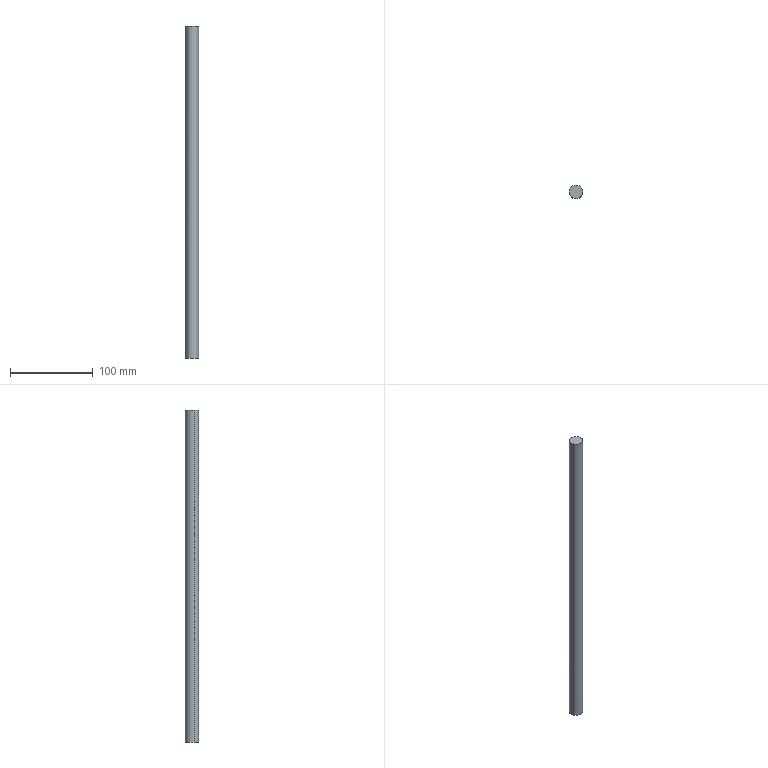Component | SolidWorks | CSFA2082 078-5 | 1 solid | 4 faces | box 16 x 16 x 400 mm | volume 80425 mm3 | cylinder 2 | plane 2 | commonest cylinder face diameters 16 x2
build123d program:
from build123d import *

# Parameters (mm, degrees)
SKETCH1_R      = 8
EXTRUDE1_DEPTH = 400


with BuildPart() as part:
    # Sketch1 → Extrude1 (new body)
    with BuildSketch(Plane.XY):
        Circle(SKETCH1_R)
    extrude(amount=EXTRUDE1_DEPTH)


solid = part.part

# Placed as in the assembly
solid = solid.moved(Location((-337.449, -241.176, 87), (0, 0, 0)))
STEP:
#1=CARTESIAN_POINT('',(-12.989,-9.387,19.173));
#2=VERTEX_POINT('',#1);
#3=CARTESIAN_POINT('',(-13.581,-9.603,19.173));
#4=VERTEX_POINT('',#3);
#5=CARTESIAN_POINT('',(-13.285,-9.495,19.173));
#6=DIRECTION('',(0.,0.,1.));
#7=DIRECTION('',(0.9395,0.3426,0.));
#8=AXIS2_PLACEMENT_3D('',#5,#6,#7);
#9=CIRCLE('',#8,0.315);
#10=EDGE_CURVE('',#2,#4,#9,.T.);
#11=ORIENTED_EDGE('',*,*,#10,.F.);
#12=CARTESIAN_POINT('',(-12.989,-9.387,3.425));
#13=VERTEX_POINT('',#12);
#14=CARTESIAN_POINT('',(-12.989,-9.387,19.173));
#15=DIRECTION('',(0.,0.,-1.));
#16=VECTOR('',#15,39.37);
#17=LINE('',#14,#16);
#18=EDGE_CURVE('',#2,#13,#17,.T.);
#19=ORIENTED_EDGE('',*,*,#18,.T.);
#20=CARTESIAN_POINT('',(-13.581,-9.603,3.425));
#21=VERTEX_POINT('',#20);
#22=CARTESIAN_POINT('',(-13.285,-9.495,3.425));
#23=DIRECTION('',(0.,0.,1.));
#24=DIRECTION('',(0.9395,0.3426,0.));
#25=AXIS2_PLACEMENT_3D('',#22,#23,#24);
#26=CIRCLE('',#25,0.315);
#27=EDGE_CURVE('',#13,#21,#26,.T.);
#28=ORIENTED_EDGE('',*,*,#27,.T.);
#29=CARTESIAN_POINT('',(-13.581,-9.603,19.173));
#30=DIRECTION('',(0.,0.,-1.));
#31=VECTOR('',#30,39.37);
#32=LINE('',#29,#31);
#33=EDGE_CURVE('',#4,#21,#32,.T.);
#34=ORIENTED_EDGE('',*,*,#33,.F.);
#35=EDGE_LOOP('',(#11,#19,#28,#34));
#36=FACE_OUTER_BOUND('',#35,.T.);
#37=CARTESIAN_POINT('',(-13.285,-9.495,19.173));
#38=DIRECTION('',(0.,0.,-1.));
#39=DIRECTION('',(-0.9395,-0.3426,0.));
#40=AXIS2_PLACEMENT_3D('',#37,#38,#39);
#41=CYLINDRICAL_SURFACE('',#40,0.315);
#42=ADVANCED_FACE('',(#36),#41,.T.);
#43=ORIENTED_EDGE('',*,*,#18,.F.);
#44=CARTESIAN_POINT('',(-13.285,-9.495,19.173));
#45=DIRECTION('',(0.,0.,1.));
#46=DIRECTION('',(0.9395,0.3426,0.));
#47=AXIS2_PLACEMENT_3D('',#44,#45,#46);
#48=CIRCLE('',#47,0.315);
#49=EDGE_CURVE('',#4,#2,#48,.T.);
#50=ORIENTED_EDGE('',*,*,#49,.F.);
#51=ORIENTED_EDGE('',*,*,#33,.T.);
#52=CARTESIAN_POINT('',(-13.285,-9.495,3.425));
#53=DIRECTION('',(0.,0.,1.));
#54=DIRECTION('',(0.9395,0.3426,0.));
#55=AXIS2_PLACEMENT_3D('',#52,#53,#54);
#56=CIRCLE('',#55,0.315);
#57=EDGE_CURVE('',#21,#13,#56,.T.);
#58=ORIENTED_EDGE('',*,*,#57,.T.);
#59=EDGE_LOOP('',(#43,#50,#51,#58));
#60=FACE_OUTER_BOUND('',#59,.T.);
#61=CARTESIAN_POINT('',(-13.285,-9.495,19.173));
#62=DIRECTION('',(0.,0.,-1.));
#63=DIRECTION('',(-0.9395,-0.3426,0.));
#64=AXIS2_PLACEMENT_3D('',#61,#62,#63);
#65=CYLINDRICAL_SURFACE('',#64,0.315);
#66=ADVANCED_FACE('',(#60),#65,.T.);
#67=ORIENTED_EDGE('',*,*,#49,.T.);
#68=ORIENTED_EDGE('',*,*,#10,.T.);
#69=EDGE_LOOP('',(#67,#68));
#70=FACE_OUTER_BOUND('',#69,.T.);
#71=CARTESIAN_POINT('',(-13.285,-9.495,19.173));
#72=DIRECTION('',(0.,0.,1.));
#73=DIRECTION('',(0.9395,0.3426,0.));
#74=AXIS2_PLACEMENT_3D('',#71,#72,#73);
#75=PLANE('',#74);
#76=ADVANCED_FACE('',(#70),#75,.T.);
#77=ORIENTED_EDGE('',*,*,#57,.F.);
#78=ORIENTED_EDGE('',*,*,#27,.F.);
#79=EDGE_LOOP('',(#77,#78));
#80=FACE_OUTER_BOUND('',#79,.T.);
#81=CARTESIAN_POINT('',(-13.285,-9.495,3.425));
#82=DIRECTION('',(0.,0.,1.));
#83=DIRECTION('',(0.9395,0.3426,0.));
#84=AXIS2_PLACEMENT_3D('',#81,#82,#83);
#85=PLANE('',#84);
#86=ADVANCED_FACE('',(#80),#85,.F.);
#87=CLOSED_SHELL('',(#42,#66,#76,#86));
#88=MANIFOLD_SOLID_BREP('',#87);
#89=CARTESIAN_POINT('',(0.,0.,0.));
#90=DIRECTION('',(0.,0.,1.));
#91=DIRECTION('',(1.,0.,0.));
#92=AXIS2_PLACEMENT_3D('',#89,#90,#91);
#93=(LENGTH_UNIT()NAMED_UNIT(*)SI_UNIT($,.METRE.));
#94=LENGTH_MEASURE_WITH_UNIT(LENGTH_MEASURE(0.0254),#93);
#95=DIMENSIONAL_EXPONENTS(1.,0.,0.,0.,0.,0.,0.);
#96=(CONVERSION_BASED_UNIT('',#94)LENGTH_UNIT()NAMED_UNIT(#95));
#97=UNCERTAINTY_MEASURE_WITH_UNIT(LENGTH_MEASURE(0.00001),#96,'','');
#98=(NAMED_UNIT(*)PLANE_ANGLE_UNIT()SI_UNIT($,.RADIAN.));
#99=(NAMED_UNIT(*)SI_UNIT($,.STERADIAN.)SOLID_ANGLE_UNIT());
#100=(GEOMETRIC_REPRESENTATION_CONTEXT(3)GLOBAL_UNCERTAINTY_ASSIGNED_CONTEXT((#97))GLOBAL_UNIT_ASSIGNED_CONTEXT((#96,#98,#99))REPRESENTATION_CONTEXT('',''));
#101=ADVANCED_BREP_SHAPE_REPRESENTATION('',(#88,#92),#100);
#102=COLOUR_RGB('',0.7922,0.8196,0.9333);
#103=FILL_AREA_STYLE_COLOUR('',#102);
#104=FILL_AREA_STYLE('',(#103));
#105=SURFACE_STYLE_FILL_AREA(#104);
#106=SURFACE_SIDE_STYLE('',(#105));
#107=SURFACE_STYLE_USAGE(.BOTH.,#106);
#108=PRESENTATION_STYLE_ASSIGNMENT((#107));
#109=STYLED_ITEM('',(#108),#88);
#110=(LENGTH_UNIT()NAMED_UNIT(*)SI_UNIT($,.METRE.));
#111=LENGTH_MEASURE_WITH_UNIT(LENGTH_MEASURE(0.0254),#110);
#112=DIMENSIONAL_EXPONENTS(1.,0.,0.,0.,0.,0.,0.);
#113=(CONVERSION_BASED_UNIT('',#111)LENGTH_UNIT()NAMED_UNIT(#112));
#114=UNCERTAINTY_MEASURE_WITH_UNIT(LENGTH_MEASURE(0.00001),#113,'','');
#115=(NAMED_UNIT(*)PLANE_ANGLE_UNIT()SI_UNIT($,.RADIAN.));
#116=(NAMED_UNIT(*)SI_UNIT($,.STERADIAN.)SOLID_ANGLE_UNIT());
#117=(GEOMETRIC_REPRESENTATION_CONTEXT(3)GLOBAL_UNCERTAINTY_ASSIGNED_CONTEXT((#114))GLOBAL_UNIT_ASSIGNED_CONTEXT((#113,#115,#116))REPRESENTATION_CONTEXT('',''));
#118=MECHANICAL_DESIGN_GEOMETRIC_PRESENTATION_REPRESENTATION('',(#109),#117);
#119=PRESENTATION_LAYER_ASSIGNMENT('','',(#109));